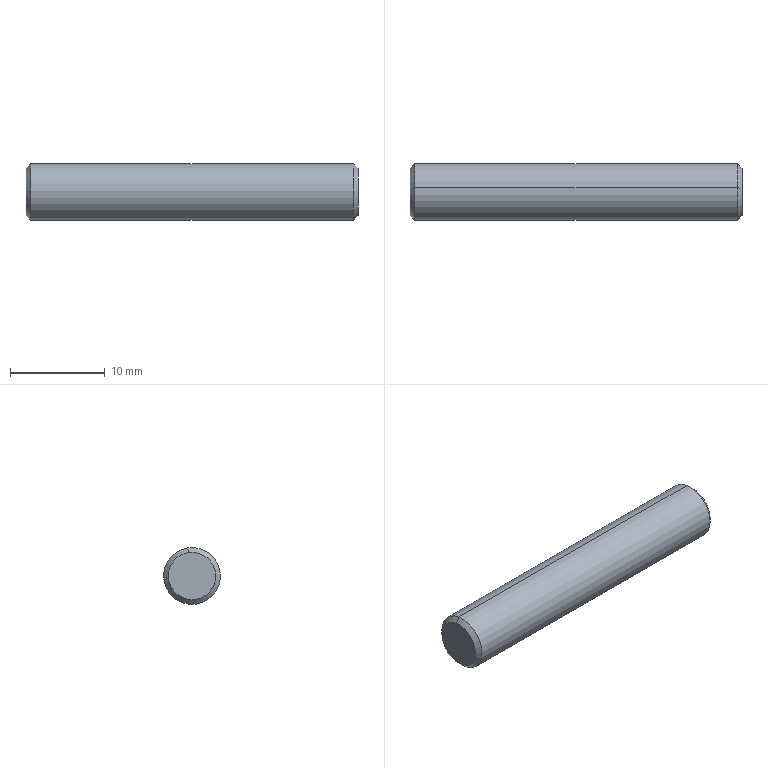Component | SolidWorks | LowerSideBeltXG-XG1-1_6Pin-1 | 1 solid | 8 faces | box 35 x 6 x 6 mm | volume 985 mm3 | cone 4 | cylinder 2 | plane 2 | commonest cylinder face diameters 6 x2
build123d program:
from build123d import *

# Parameters (mm, degrees)
SKETCH1_R           = 3
BOSS_EXTRUDE1_DEPTH = 35
CHAMFER1_SIZE       = 0.5


with BuildPart() as part:
    # Sketch1 → Boss-Extrude1 (new body)
    with BuildSketch(Plane.XY):
        Circle(SKETCH1_R)
    extrude(amount=BOSS_EXTRUDE1_DEPTH)

    # Chamfer1
    chamfer1_edges = [part.edges().sort_by_distance(p)[0] for p in [
        (-3, 0, 0),
        (-3, 0, 35),
    ]]
    chamfer(chamfer1_edges, length=CHAMFER1_SIZE)


solid = part.part

# Placed as in the assembly
solid = solid.moved(Location((-194.22, 625, 114), (0, 90, 0)))
STEP:
#1=COLOUR_RGB('',0.7922,0.8196,0.9333);
#2=FILL_AREA_STYLE_COLOUR('',#1);
#3=FILL_AREA_STYLE('',(#2));
#4=SURFACE_STYLE_FILL_AREA(#3);
#5=SURFACE_SIDE_STYLE('',(#4));
#6=SURFACE_STYLE_USAGE(.BOTH.,#5);
#7=PRESENTATION_STYLE_ASSIGNMENT((#6));
#8=CARTESIAN_POINT('',(-6.268,24.621,4.585));
#9=VERTEX_POINT('',#8);
#10=CARTESIAN_POINT('',(-6.268,24.592,4.391));
#11=VERTEX_POINT('',#10);
#12=CARTESIAN_POINT('',(-6.268,24.606,4.488));
#13=DIRECTION('',(1.,0.,0.));
#14=DIRECTION('',(0.,0.1502,0.9887));
#15=AXIS2_PLACEMENT_3D('',#12,#13,#14);
#16=CIRCLE('',#15,0.09843);
#17=EDGE_CURVE('',#9,#11,#16,.T.);
#18=ORIENTED_EDGE('',*,*,#17,.F.);
#19=CARTESIAN_POINT('',(-6.288,24.624,4.605));
#20=VERTEX_POINT('',#19);
#21=CARTESIAN_POINT('',(-6.268,24.621,4.585));
#22=DIRECTION('',(-0.7071,0.1062,0.6991));
#23=VECTOR('',#22,39.37);
#24=LINE('',#21,#23);
#25=EDGE_CURVE('',#9,#20,#24,.T.);
#26=ORIENTED_EDGE('',*,*,#25,.T.);
#27=CARTESIAN_POINT('',(-6.288,24.589,4.371));
#28=VERTEX_POINT('',#27);
#29=CARTESIAN_POINT('',(-6.288,24.606,4.488));
#30=DIRECTION('',(-1.,-0.,-0.));
#31=DIRECTION('',(0.,0.1502,0.9887));
#32=AXIS2_PLACEMENT_3D('',#29,#30,#31);
#33=CIRCLE('',#32,0.1181);
#34=EDGE_CURVE('',#28,#20,#33,.T.);
#35=ORIENTED_EDGE('',*,*,#34,.F.);
#36=CARTESIAN_POINT('',(-6.268,24.592,4.391));
#37=DIRECTION('',(-0.7071,-0.1062,-0.6991));
#38=VECTOR('',#37,39.37);
#39=LINE('',#36,#38);
#40=EDGE_CURVE('',#11,#28,#39,.T.);
#41=ORIENTED_EDGE('',*,*,#40,.F.);
#42=EDGE_LOOP('',(#18,#26,#35,#41));
#43=FACE_OUTER_BOUND('',#42,.T.);
#44=CARTESIAN_POINT('',(-6.268,24.606,4.488));
#45=DIRECTION('',(-1.,-0.,-0.));
#46=DIRECTION('',(0.,-0.1502,-0.9887));
#47=AXIS2_PLACEMENT_3D('',#44,#45,#46);
#48=CONICAL_SURFACE('',#47,0.09843,0.7854);
#49=ADVANCED_FACE('',(#43),#48,.T.);
#50=CARTESIAN_POINT('',(-7.646,24.592,4.391));
#51=VERTEX_POINT('',#50);
#52=CARTESIAN_POINT('',(-7.646,24.621,4.585));
#53=VERTEX_POINT('',#52);
#54=CARTESIAN_POINT('',(-7.646,24.606,4.488));
#55=DIRECTION('',(-1.,-0.,-0.));
#56=DIRECTION('',(0.,0.1502,0.9887));
#57=AXIS2_PLACEMENT_3D('',#54,#55,#56);
#58=CIRCLE('',#57,0.09843);
#59=EDGE_CURVE('',#51,#53,#58,.T.);
#60=ORIENTED_EDGE('',*,*,#59,.F.);
#61=CARTESIAN_POINT('',(-7.627,24.589,4.371));
#62=VERTEX_POINT('',#61);
#63=CARTESIAN_POINT('',(-7.627,24.589,4.371));
#64=DIRECTION('',(0.7071,-0.1062,-0.6991));
#65=VECTOR('',#64,39.37);
#66=LINE('',#63,#65);
#67=EDGE_CURVE('',#51,#62,#66,.T.);
#68=ORIENTED_EDGE('',*,*,#67,.T.);
#69=CARTESIAN_POINT('',(-7.627,24.624,4.605));
#70=VERTEX_POINT('',#69);
#71=CARTESIAN_POINT('',(-7.627,24.606,4.488));
#72=DIRECTION('',(1.,0.,0.));
#73=DIRECTION('',(0.,0.1502,0.9887));
#74=AXIS2_PLACEMENT_3D('',#71,#72,#73);
#75=CIRCLE('',#74,0.1181);
#76=EDGE_CURVE('',#70,#62,#75,.T.);
#77=ORIENTED_EDGE('',*,*,#76,.F.);
#78=CARTESIAN_POINT('',(-7.627,24.624,4.605));
#79=DIRECTION('',(0.7071,0.1062,0.6991));
#80=VECTOR('',#79,39.37);
#81=LINE('',#78,#80);
#82=EDGE_CURVE('',#53,#70,#81,.T.);
#83=ORIENTED_EDGE('',*,*,#82,.F.);
#84=EDGE_LOOP('',(#60,#68,#77,#83));
#85=FACE_OUTER_BOUND('',#84,.T.);
#86=CARTESIAN_POINT('',(-7.627,24.606,4.488));
#87=DIRECTION('',(1.,0.,0.));
#88=DIRECTION('',(0.,0.1502,0.9887));
#89=AXIS2_PLACEMENT_3D('',#86,#87,#88);
#90=CONICAL_SURFACE('',#89,0.1181,0.7854);
#91=ADVANCED_FACE('',(#85),#90,.T.);
#92=ORIENTED_EDGE('',*,*,#34,.T.);
#93=CARTESIAN_POINT('',(-6.268,24.624,4.605));
#94=DIRECTION('',(-1.,-0.,-0.));
#95=VECTOR('',#94,39.37);
#96=LINE('',#93,#95);
#97=EDGE_CURVE('',#20,#70,#96,.T.);
#98=ORIENTED_EDGE('',*,*,#97,.T.);
#99=ORIENTED_EDGE('',*,*,#76,.T.);
#100=CARTESIAN_POINT('',(-6.268,24.589,4.371));
#101=DIRECTION('',(-1.,-0.,-0.));
#102=VECTOR('',#101,39.37);
#103=LINE('',#100,#102);
#104=EDGE_CURVE('',#28,#62,#103,.T.);
#105=ORIENTED_EDGE('',*,*,#104,.F.);
#106=EDGE_LOOP('',(#92,#98,#99,#105));
#107=FACE_OUTER_BOUND('',#106,.T.);
#108=CARTESIAN_POINT('',(-6.268,24.606,4.488));
#109=DIRECTION('',(-1.,-0.,-0.));
#110=DIRECTION('',(0.,-0.1502,-0.9887));
#111=AXIS2_PLACEMENT_3D('',#108,#109,#110);
#112=CYLINDRICAL_SURFACE('',#111,0.1181);
#113=ADVANCED_FACE('',(#107),#112,.T.);
#114=ORIENTED_EDGE('',*,*,#97,.F.);
#115=CARTESIAN_POINT('',(-6.288,24.606,4.488));
#116=DIRECTION('',(-1.,-0.,-0.));
#117=DIRECTION('',(0.,0.1502,0.9887));
#118=AXIS2_PLACEMENT_3D('',#115,#116,#117);
#119=CIRCLE('',#118,0.1181);
#120=EDGE_CURVE('',#20,#28,#119,.T.);
#121=ORIENTED_EDGE('',*,*,#120,.T.);
#122=ORIENTED_EDGE('',*,*,#104,.T.);
#123=CARTESIAN_POINT('',(-7.627,24.606,4.488));
#124=DIRECTION('',(1.,0.,0.));
#125=DIRECTION('',(0.,0.1502,0.9887));
#126=AXIS2_PLACEMENT_3D('',#123,#124,#125);
#127=CIRCLE('',#126,0.1181);
#128=EDGE_CURVE('',#62,#70,#127,.T.);
#129=ORIENTED_EDGE('',*,*,#128,.T.);
#130=EDGE_LOOP('',(#114,#121,#122,#129));
#131=FACE_OUTER_BOUND('',#130,.T.);
#132=CARTESIAN_POINT('',(-6.268,24.606,4.488));
#133=DIRECTION('',(-1.,-0.,-0.));
#134=DIRECTION('',(0.,-0.1502,-0.9887));
#135=AXIS2_PLACEMENT_3D('',#132,#133,#134);
#136=CYLINDRICAL_SURFACE('',#135,0.1181);
#137=ADVANCED_FACE('',(#131),#136,.T.);
#138=CARTESIAN_POINT('',(-6.268,24.606,4.488));
#139=DIRECTION('',(1.,0.,0.));
#140=DIRECTION('',(0.,0.1502,0.9887));
#141=AXIS2_PLACEMENT_3D('',#138,#139,#140);
#142=CIRCLE('',#141,0.09843);
#143=EDGE_CURVE('',#11,#9,#142,.T.);
#144=ORIENTED_EDGE('',*,*,#143,.T.);
#145=ORIENTED_EDGE('',*,*,#17,.T.);
#146=EDGE_LOOP('',(#144,#145));
#147=FACE_OUTER_BOUND('',#146,.T.);
#148=CARTESIAN_POINT('',(-6.268,24.606,4.488));
#149=DIRECTION('',(1.,0.,0.));
#150=DIRECTION('',(-0.,0.1502,0.9887));
#151=AXIS2_PLACEMENT_3D('',#148,#149,#150);
#152=PLANE('',#151);
#153=ADVANCED_FACE('',(#147),#152,.T.);
#154=CARTESIAN_POINT('',(-7.646,24.606,4.488));
#155=DIRECTION('',(-1.,-0.,-0.));
#156=DIRECTION('',(0.,0.1502,0.9887));
#157=AXIS2_PLACEMENT_3D('',#154,#155,#156);
#158=CIRCLE('',#157,0.09843);
#159=EDGE_CURVE('',#53,#51,#158,.T.);
#160=ORIENTED_EDGE('',*,*,#159,.T.);
#161=ORIENTED_EDGE('',*,*,#59,.T.);
#162=EDGE_LOOP('',(#160,#161));
#163=FACE_OUTER_BOUND('',#162,.T.);
#164=CARTESIAN_POINT('',(-7.646,24.606,4.488));
#165=DIRECTION('',(1.,0.,0.));
#166=DIRECTION('',(-0.,0.1502,0.9887));
#167=AXIS2_PLACEMENT_3D('',#164,#165,#166);
#168=PLANE('',#167);
#169=ADVANCED_FACE('',(#163),#168,.F.);
#170=ORIENTED_EDGE('',*,*,#67,.F.);
#171=ORIENTED_EDGE('',*,*,#159,.F.);
#172=ORIENTED_EDGE('',*,*,#82,.T.);
#173=ORIENTED_EDGE('',*,*,#128,.F.);
#174=EDGE_LOOP('',(#170,#171,#172,#173));
#175=FACE_OUTER_BOUND('',#174,.T.);
#176=CARTESIAN_POINT('',(-7.627,24.606,4.488));
#177=DIRECTION('',(1.,0.,0.));
#178=DIRECTION('',(0.,0.1502,0.9887));
#179=AXIS2_PLACEMENT_3D('',#176,#177,#178);
#180=CONICAL_SURFACE('',#179,0.1181,0.7854);
#181=ADVANCED_FACE('',(#175),#180,.T.);
#182=ORIENTED_EDGE('',*,*,#25,.F.);
#183=ORIENTED_EDGE('',*,*,#143,.F.);
#184=ORIENTED_EDGE('',*,*,#40,.T.);
#185=ORIENTED_EDGE('',*,*,#120,.F.);
#186=EDGE_LOOP('',(#182,#183,#184,#185));
#187=FACE_OUTER_BOUND('',#186,.T.);
#188=CARTESIAN_POINT('',(-6.268,24.606,4.488));
#189=DIRECTION('',(-1.,-0.,-0.));
#190=DIRECTION('',(0.,-0.1502,-0.9887));
#191=AXIS2_PLACEMENT_3D('',#188,#189,#190);
#192=CONICAL_SURFACE('',#191,0.09843,0.7854);
#193=ADVANCED_FACE('',(#187),#192,.T.);
#194=CLOSED_SHELL('',(#49,#91,#113,#137,#153,#169,#181,#193));
#195=MANIFOLD_SOLID_BREP('',#194);
#196=STYLED_ITEM('',(#7),#195);
#197=PRESENTATION_LAYER_ASSIGNMENT('','',(#196));
#198=CARTESIAN_POINT('',(0.,0.,0.));
#199=DIRECTION('',(0.,0.,1.));
#200=DIRECTION('',(1.,0.,0.));
#201=AXIS2_PLACEMENT_3D('',#198,#199,#200);
#202=(LENGTH_UNIT()NAMED_UNIT(*)SI_UNIT($,.METRE.));
#203=LENGTH_MEASURE_WITH_UNIT(LENGTH_MEASURE(0.0254),#202);
#204=DIMENSIONAL_EXPONENTS(1.,0.,0.,0.,0.,0.,0.);
#205=(CONVERSION_BASED_UNIT('',#203)LENGTH_UNIT()NAMED_UNIT(#204));
#206=UNCERTAINTY_MEASURE_WITH_UNIT(LENGTH_MEASURE(0.00001),#205,'','');
#207=(NAMED_UNIT(*)PLANE_ANGLE_UNIT()SI_UNIT($,.RADIAN.));
#208=(NAMED_UNIT(*)SI_UNIT($,.STERADIAN.)SOLID_ANGLE_UNIT());
#209=(GEOMETRIC_REPRESENTATION_CONTEXT(3)GLOBAL_UNCERTAINTY_ASSIGNED_CONTEXT((#206))GLOBAL_UNIT_ASSIGNED_CONTEXT((#205,#207,#208))REPRESENTATION_CONTEXT('',''));
#210=ADVANCED_BREP_SHAPE_REPRESENTATION('',(#195,#201),#209);
#211=(LENGTH_UNIT()NAMED_UNIT(*)SI_UNIT($,.METRE.));
#212=LENGTH_MEASURE_WITH_UNIT(LENGTH_MEASURE(0.0254),#211);
#213=DIMENSIONAL_EXPONENTS(1.,0.,0.,0.,0.,0.,0.);
#214=(CONVERSION_BASED_UNIT('',#212)LENGTH_UNIT()NAMED_UNIT(#213));
#215=UNCERTAINTY_MEASURE_WITH_UNIT(LENGTH_MEASURE(0.00001),#214,'','');
#216=(NAMED_UNIT(*)PLANE_ANGLE_UNIT()SI_UNIT($,.RADIAN.));
#217=(NAMED_UNIT(*)SI_UNIT($,.STERADIAN.)SOLID_ANGLE_UNIT());
#218=(GEOMETRIC_REPRESENTATION_CONTEXT(3)GLOBAL_UNCERTAINTY_ASSIGNED_CONTEXT((#215))GLOBAL_UNIT_ASSIGNED_CONTEXT((#214,#216,#217))REPRESENTATION_CONTEXT('',''));
#219=MECHANICAL_DESIGN_GEOMETRIC_PRESENTATION_REPRESENTATION('',(#196),#218);